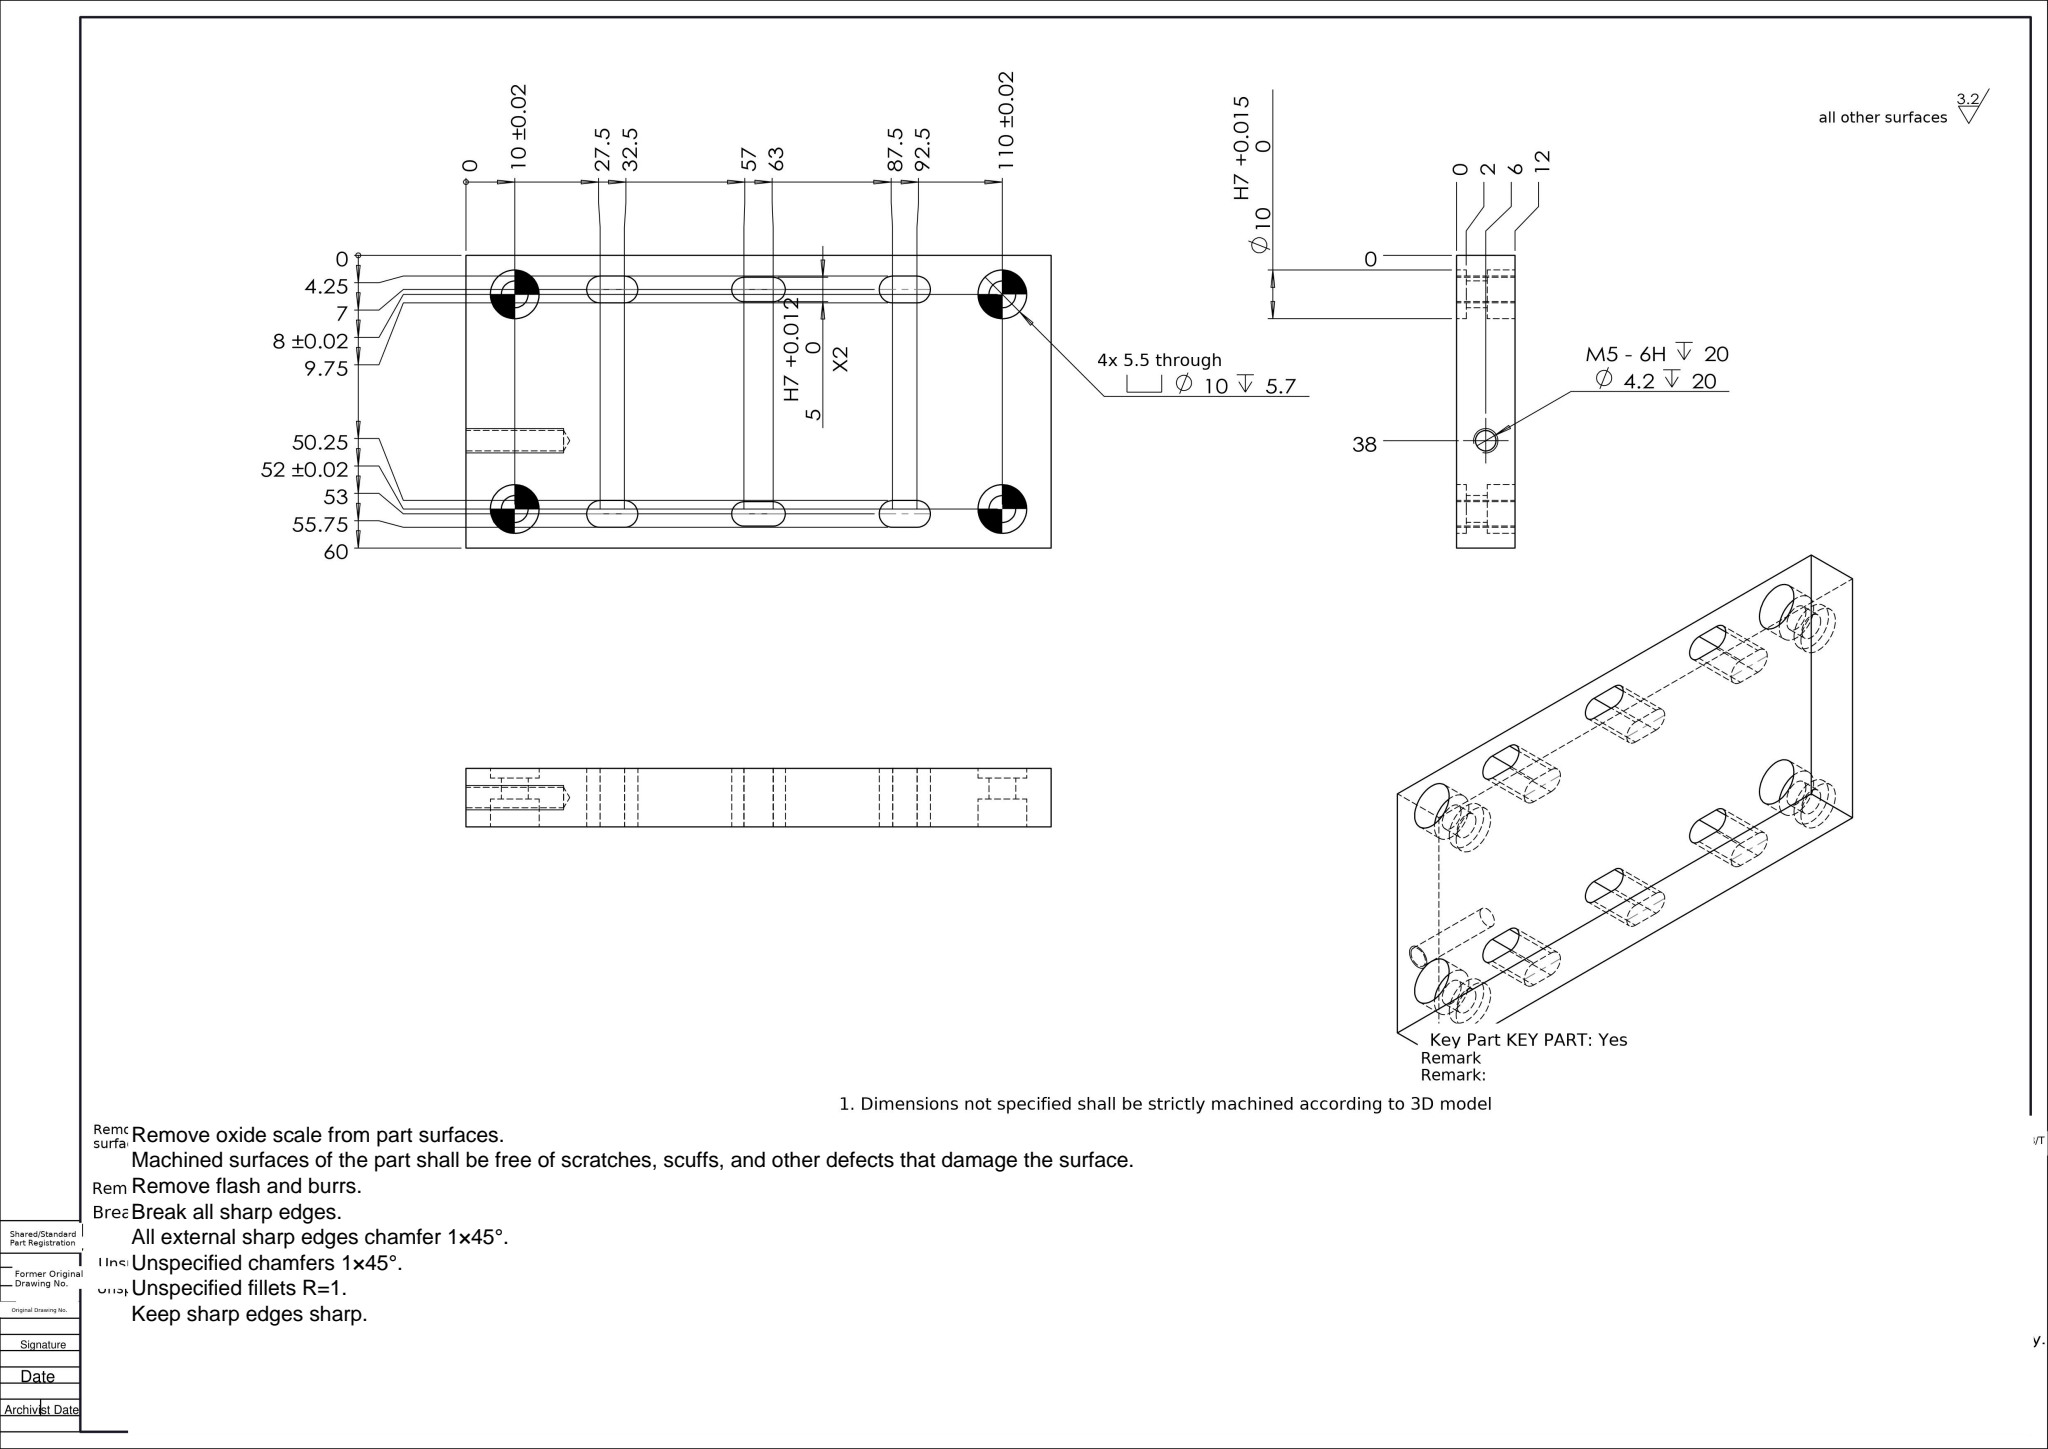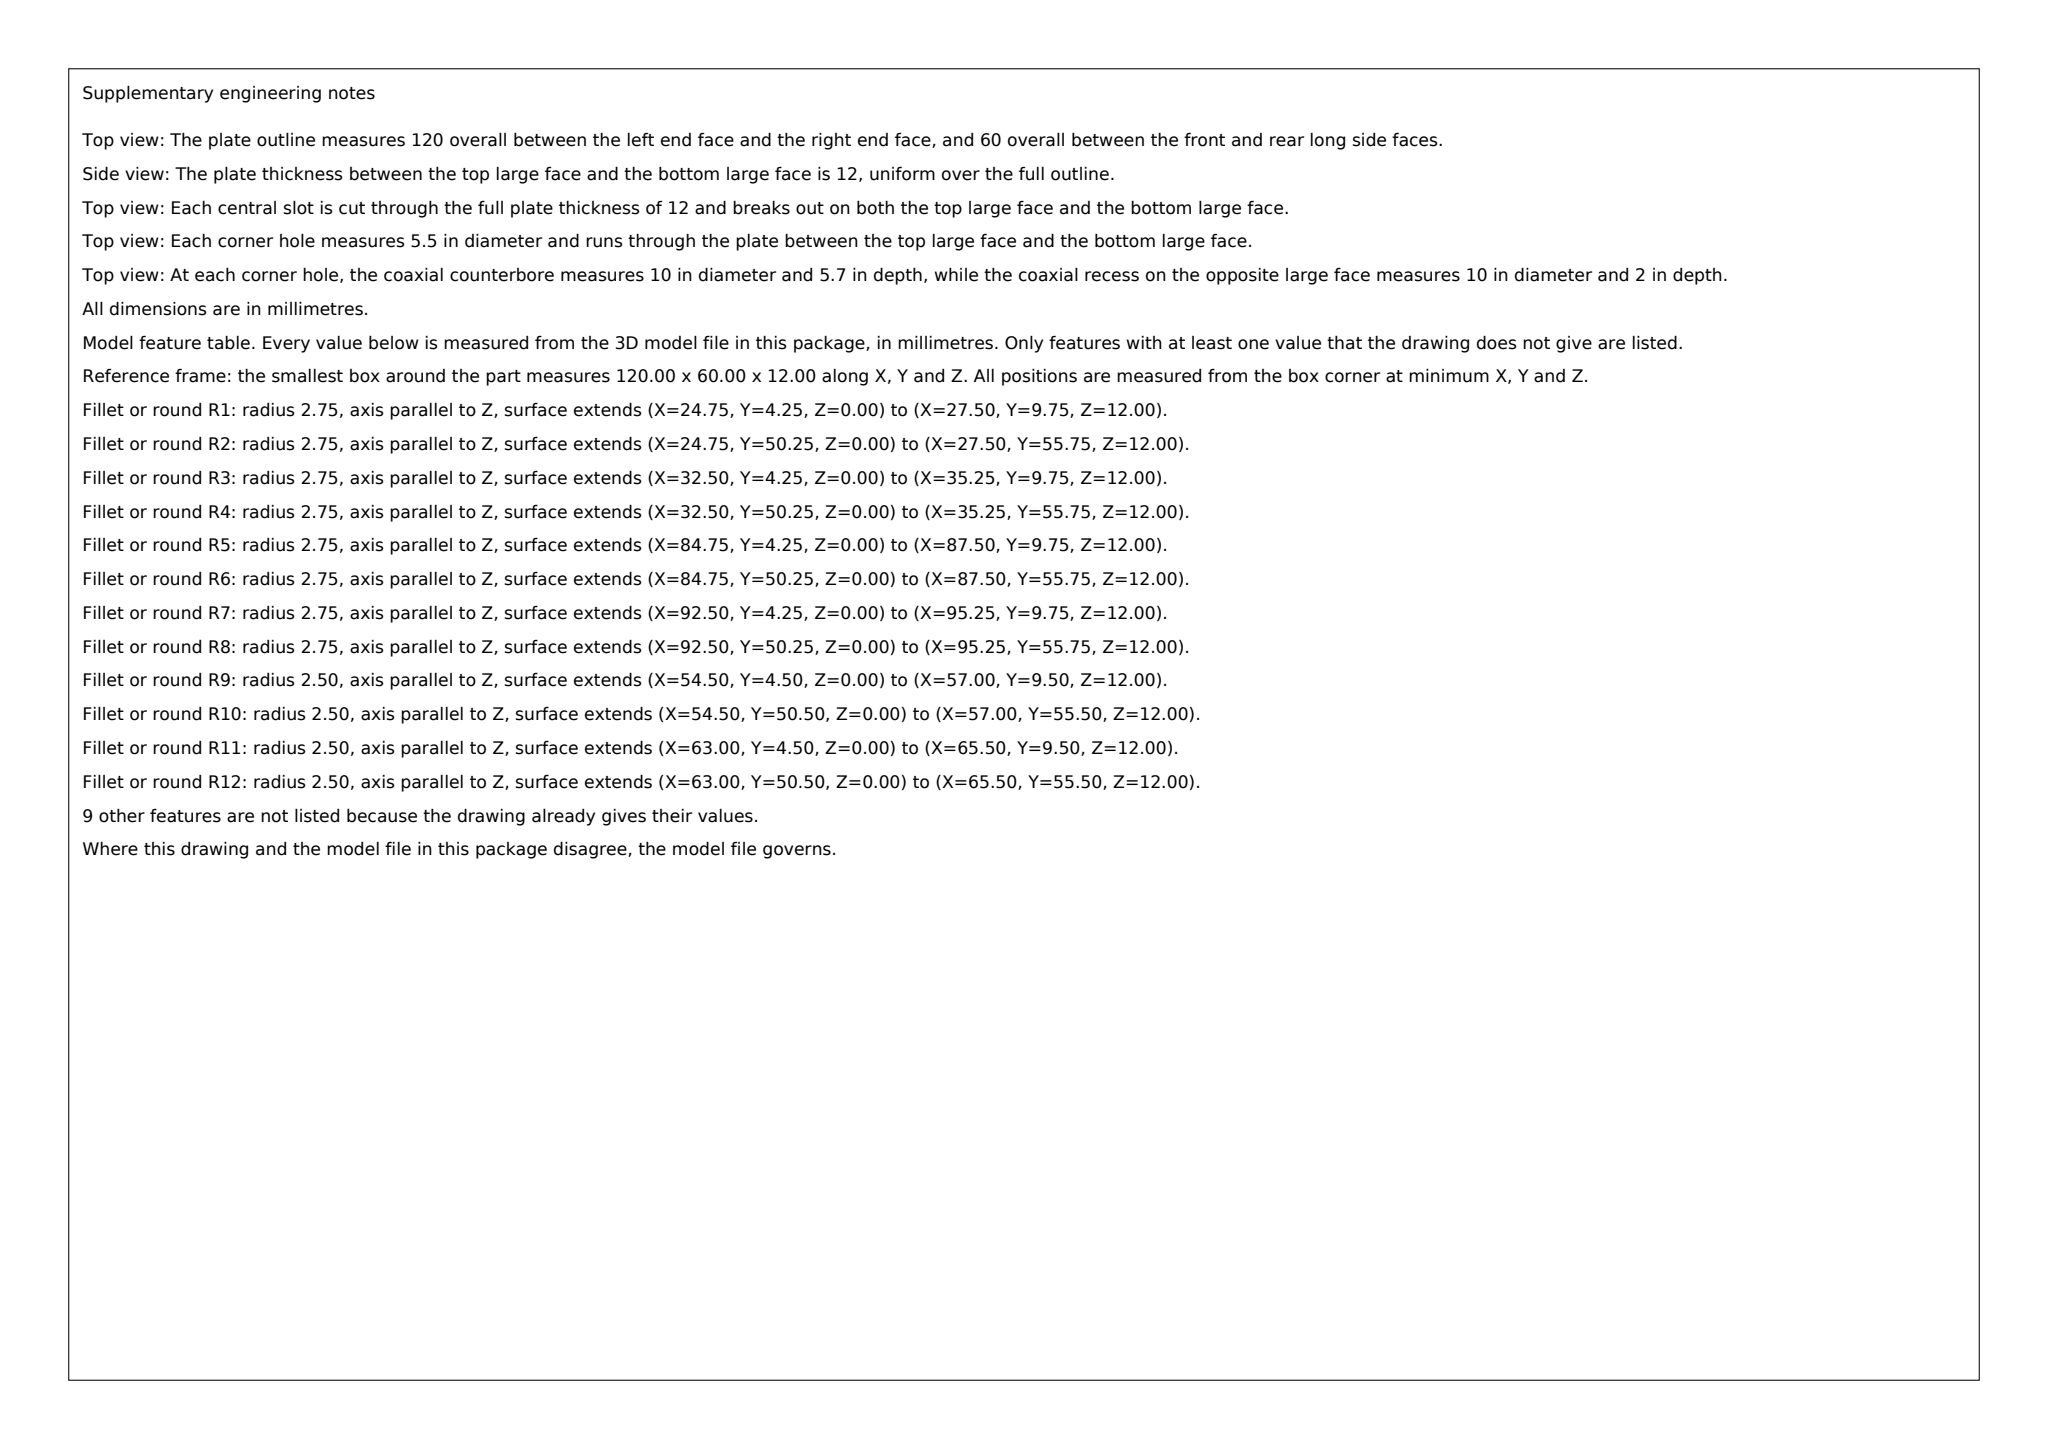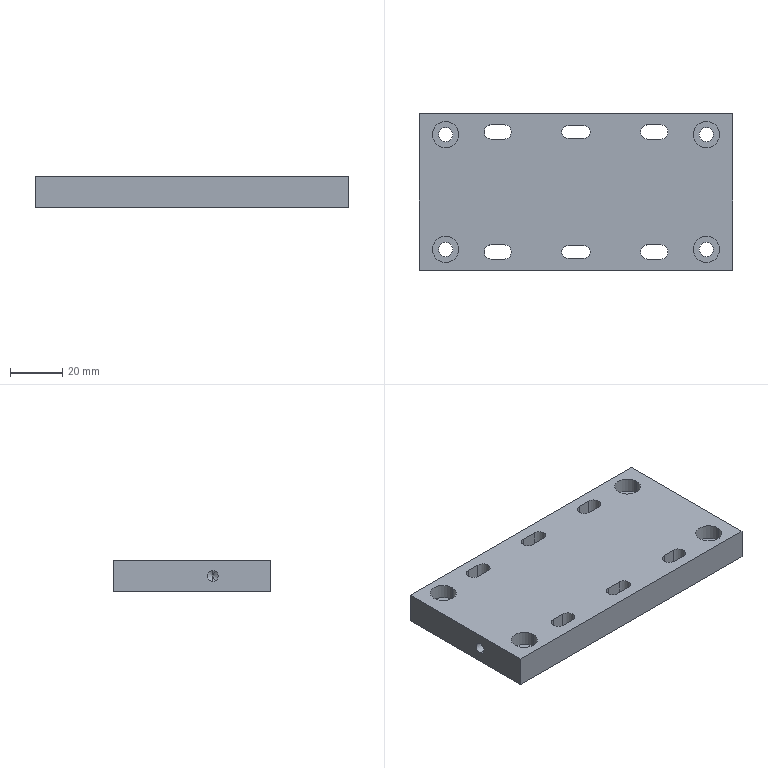Part | SolidWorks | mm | 1 solid | 72 faces | box 120 x 60 x 12 mm | volume 79638 mm3 | cylinder 44 | plane 26 | cone 2 | commonest cylinder face diameters 5.5 x20 10 x16 5 x6 4.2 x2
Drawing notes:
OVERALL PLATE 120 x 60 x 12 THK; Ø10 H7 bore centres at X=10 and X=110 from left edge give 10 mm edge distance at each end. | from the solid: bbox_xyz [120.0, 60.0, 12.0]; planes x=0.0 and x=120.0; Ø10 cylinders at x=10.0 and x=110.0
4X OBROUND SLOT, WIDTH 5.5, END CENTRES X=27.5/32.5 AND X=87.5/92.5, AT Y=7 AND Y=53 - THRU 12. | from the solid: cylinders dia 5.5 axis z at [27.5,7],[32.5,7],[27.5,53],[32.5,53],[87.5,7],[92.5,7],[87.5,53],[92.5,53], length 12.0 = full 12 thickness
2X OBROUND SLOT, WIDTH 5 H7, END CENTRES X=57/63, AT Y=7 AND Y=53 - THRU 12. | from the solid: cylinders dia 5.0 axis z at [57,7],[63,7],[57,53],[63,53], length 12.0 = full 12 thickness
M5-6H THD 20 DEEP (Ø4.2 DRILL 20 DEEP) IN END FACE: AXIS AT Z=6 FROM BOTTOM FACE (MID-THICKNESS OF 12) AND Y=22 FROM Y=0 EDGE; 2 PLACES, ONE IN EACH 60 mm END FACE. | from the solid: cylinders dia 4.2 axis x at [y=22.0, z=6.0], length 20.0, count 2; 118° drill point cone ref dia 4.2
build123d program:
from build123d import *

# Parameters (mm, degrees)
SKETCH1_W                                         = 120
SKETCH1_H                                         = 60
BOSS_EXTRUDE1_DEPTH                               = 12
HOLE_SIZE_ACCORDING_TO_HEXAGON_SOCKET_D           = 5.5
HOLE_SIZE_ACCORDING_TO_HEXAGON_SOCKET_CBORE_D     = 10
HOLE_SIZE_ACCORDING_TO_HEXAGON_SOCKET_CBORE_DEPTH = 5.7
CUT_EXTRUDE1_DEPTH                                = 69.147
LPATTERN1_COUNT                                   = 2
LPATTERN1_PITCH                                   = 60
LPATTERN1_COUNT_DIR2                              = 2
LPATTERN1_PITCH_DIR2                              = 46
CUT_EXTRUDE2_DEPTH                                = 12
SIZE_MM_DOWEL_PIN_HOLE_1_D                        = 10
SIZE_MM_DOWEL_PIN_HOLE_1_DEPTH                    = 2
M5_TAPPED_HOLE1_D                                 = 4.2
M5_TAPPED_HOLE1_DEPTH                             = 20
M5_TAPPED_HOLE1_TIP                               = 1.262


with BuildPart() as part:
    # Sketch1 → Boss-Extrude1 (new body)
    with BuildSketch(Plane.XY):
        Rectangle(SKETCH1_W, SKETCH1_H)
    extrude(amount=BOSS_EXTRUDE1_DEPTH)

    # Hole Size _ according to_ Hexagon Socket (through all)
    with Locations(Plane.XY.offset(12)):
        with Locations((50, 22), (50, -22), (-50, -22), (-50, 22)):
            CounterBoreHole(HOLE_SIZE_ACCORDING_TO_HEXAGON_SOCKET_D / 2, HOLE_SIZE_ACCORDING_TO_HEXAGON_SOCKET_CBORE_D / 2, HOLE_SIZE_ACCORDING_TO_HEXAGON_SOCKET_CBORE_DEPTH)

    # Sketch7 → Cut-Extrude1 (cut, through all)
    with BuildSketch(Plane(origin=(0, 0, 0), x_dir=(-1, 0, 0), z_dir=(0, 0, -1))):
        with BuildLine():
            Line((32.5, -25.75), (27.5, -25.75))
            ThreePointArc((27.5, -25.75), (24.75, -23), (27.5, -20.25))
            Line((27.5, -20.25), (32.5, -20.25))
            ThreePointArc((32.5, -20.25), (35.25, -23), (32.5, -25.75))
        make_face()
    cut_extrude1 = extrude(amount=-CUT_EXTRUDE1_DEPTH, mode=Mode.SUBTRACT)

    # LPattern1: Cut-Extrude1 2 × 2
    with Locations(*[(i * LPATTERN1_PITCH, j * LPATTERN1_PITCH_DIR2, 0) for i in range(LPATTERN1_COUNT) for j in range(LPATTERN1_COUNT_DIR2) if (i, j) != (0, 0)]):
        add(cut_extrude1, mode=Mode.SUBTRACT)

    # Sketch9 → Cut-Extrude2 (cut)
    with BuildSketch(Plane(origin=(0, 0, 0), x_dir=(-1, 0, 0), z_dir=(0, 0, -1))):
        with BuildLine():
            Line((-3, 25.5), (3, 25.5))
            ThreePointArc((3, 25.5), (5.5, 23), (3, 20.5))
            Line((3, 20.5), (-3, 20.5))
            ThreePointArc((-3, 20.5), (-5.5, 23), (-3, 25.5))
        make_face()
        with BuildLine():
            Line((-3, -20.5), (3, -20.5))
            ThreePointArc((3, -20.5), (5.5, -23), (3, -25.5))
            Line((3, -25.5), (-3, -25.5))
            ThreePointArc((-3, -25.5), (-5.5, -23), (-3, -20.5))
        make_face()
    extrude(amount=-CUT_EXTRUDE2_DEPTH, mode=Mode.SUBTRACT)

    # Size mm Dowel Pin Hole 1
    with Locations(Plane(origin=(0, 0, 0), x_dir=(-1, 0, 0), z_dir=(0, 0, -1))):
        with Locations((-50, 22), (-50, -22), (50, -22), (50, 22)):
            Hole(SIZE_MM_DOWEL_PIN_HOLE_1_D / 2, depth=SIZE_MM_DOWEL_PIN_HOLE_1_DEPTH)

    # M5 Tapped Hole1
    with Locations(Plane.ZY.offset(60)):
        with Locations((6, -8)):
            Hole(M5_TAPPED_HOLE1_D / 2, depth=M5_TAPPED_HOLE1_DEPTH)
            with Locations((0, 0, -(M5_TAPPED_HOLE1_DEPTH + M5_TAPPED_HOLE1_TIP / 2))):  # 118° drill point
                Cone(0, M5_TAPPED_HOLE1_D / 2, M5_TAPPED_HOLE1_TIP, mode=Mode.SUBTRACT)


solid = part.part